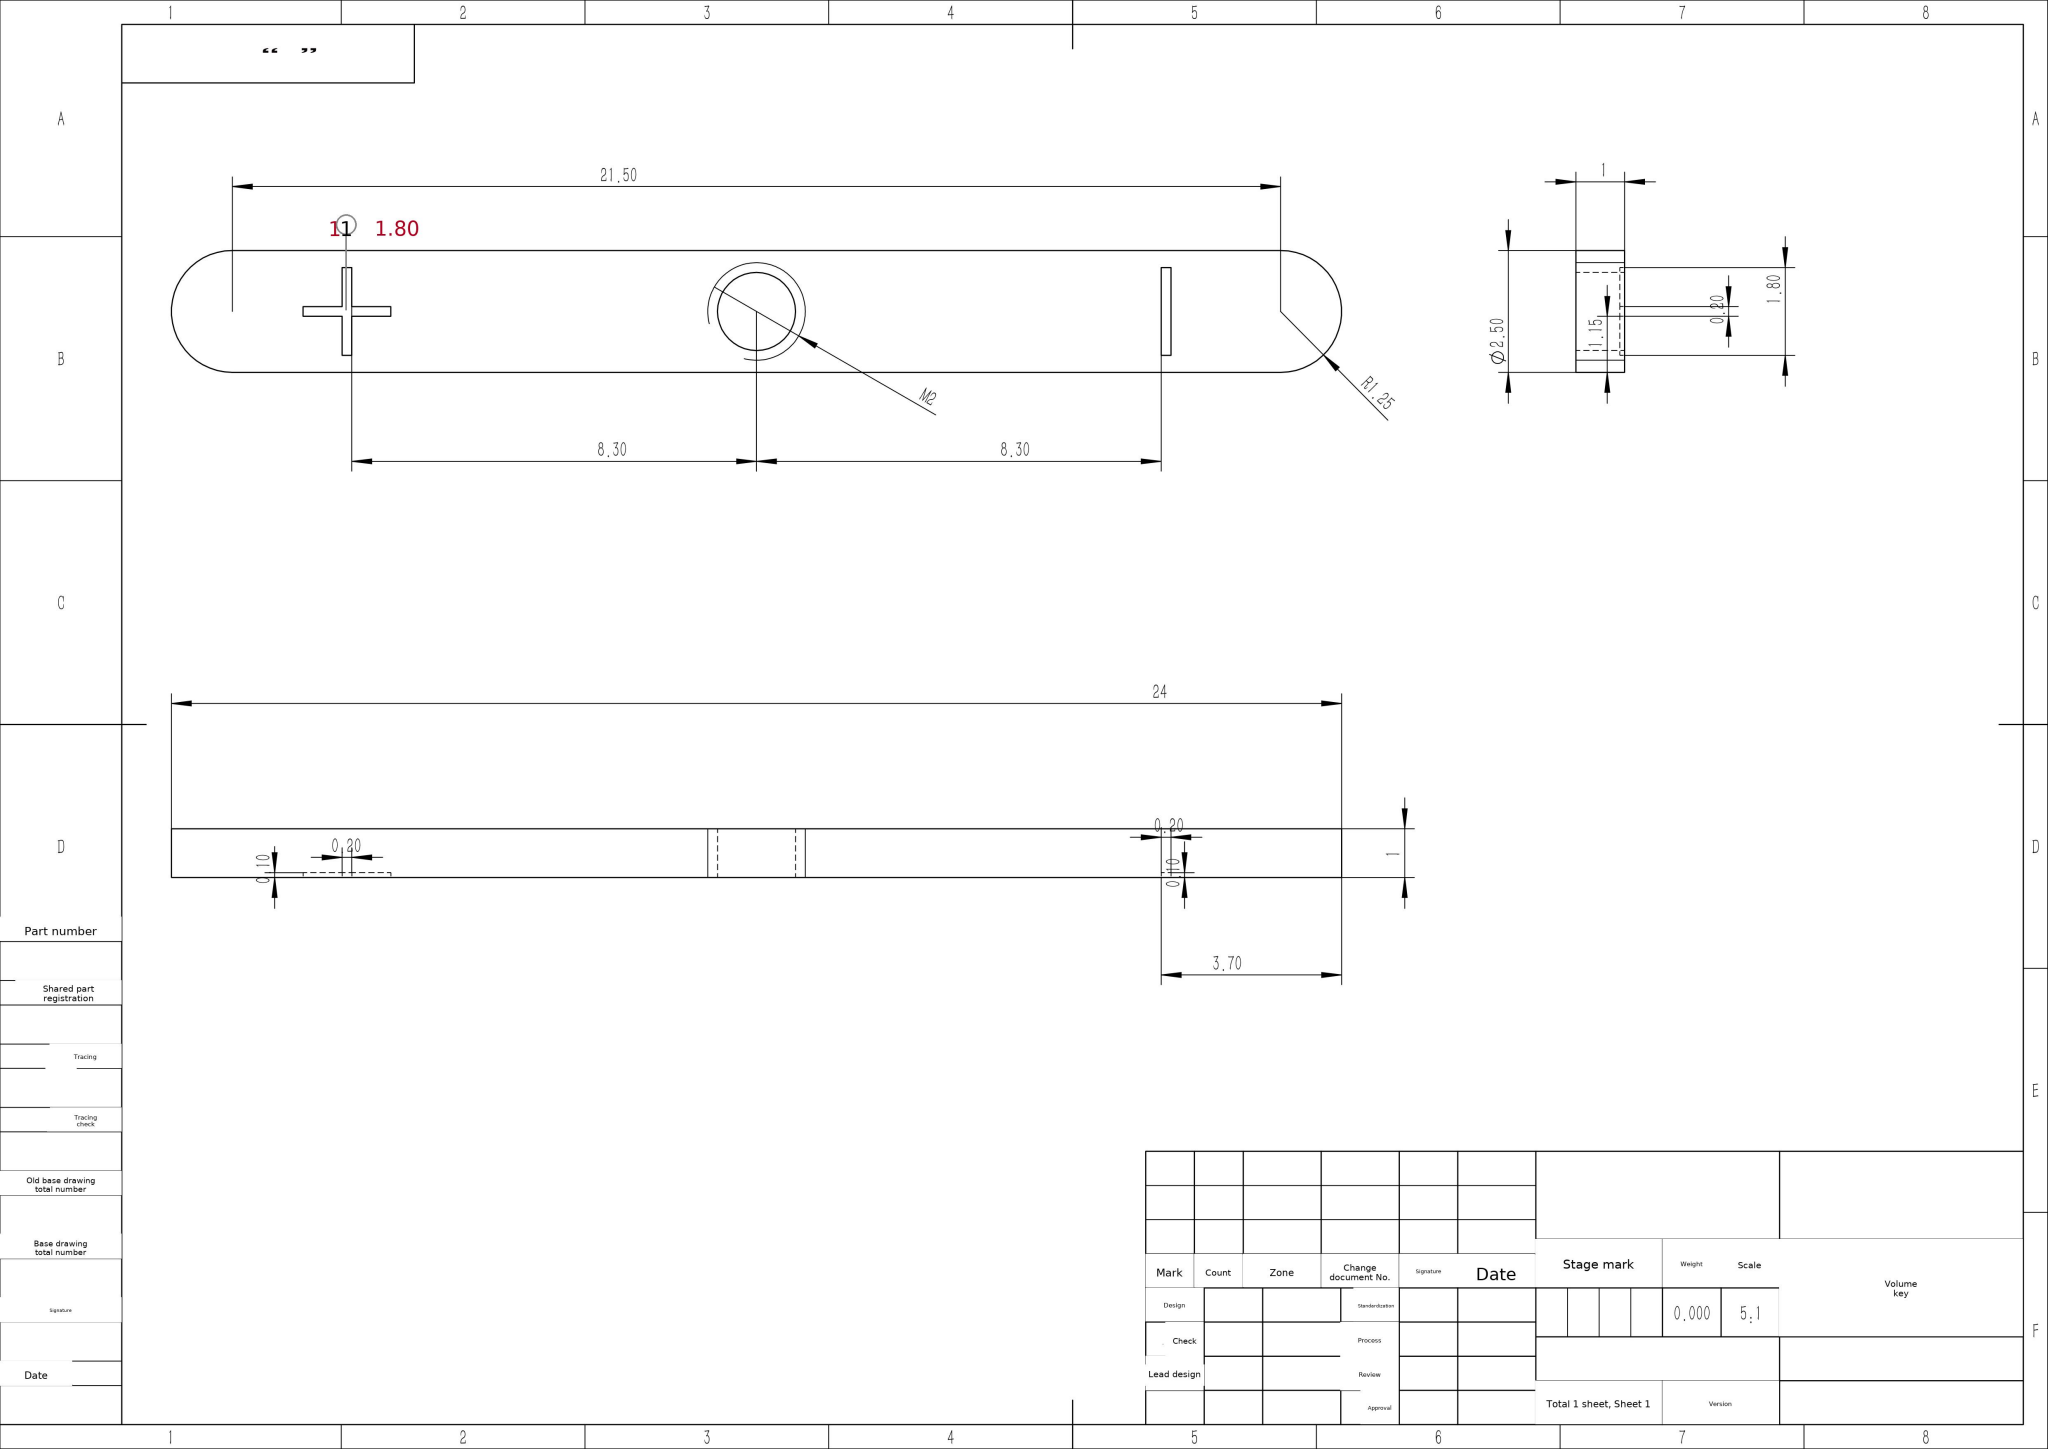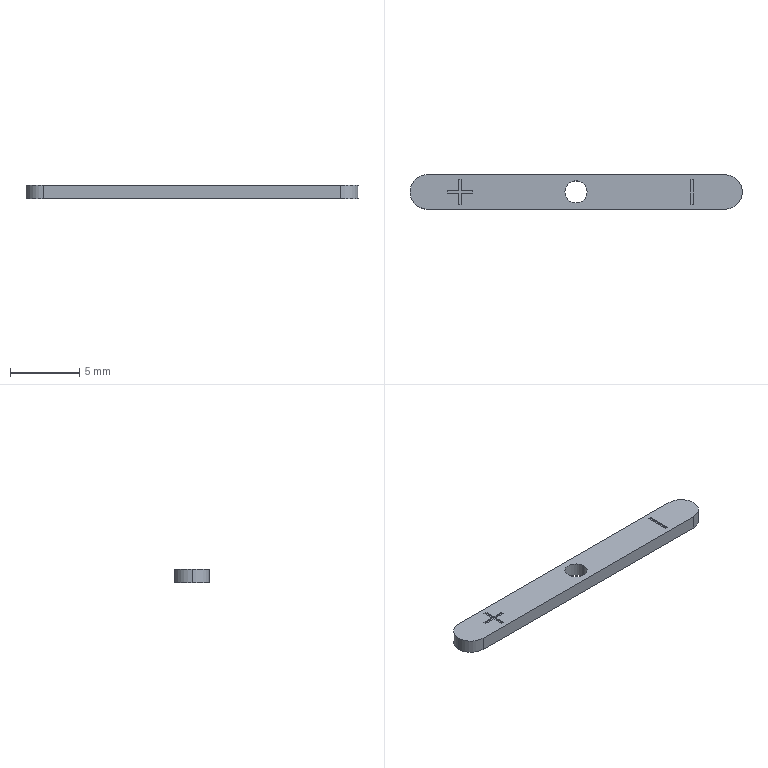Part | SolidWorks | mm | 1 solid | 27 faces | box 24 x 2.5 x 1 mm | volume 57 mm3 | plane 22 | cylinder 5 | commonest cylinder face diameters 2.5 x3 1.6 x2
build123d program:
from build123d import *

# Parameters (mm, degrees)
BOSS_EXTRUDE1_DEPTH = 1
SKETCH2_W           = 0.2
SKETCH2_H           = 1.8
SKETCH2_H_2         = 0.8
SKETCH2_W_2         = 0.8
SKETCH2_H_3         = 0.2
CUT_EXTRUDE1_DEPTH  = 0.1
M2_TAPPED_HOLE1_D   = 1.6


with BuildPart() as part:
    # Sketch1 → Boss-Extrude1 (new body)
    with BuildSketch(Plane.XY):
        with BuildLine():
            Line((-10.75, 1.25), (10.75, 1.25))
            ThreePointArc((10.75, 1.25), (12, 0), (10.75, -1.25))
            Line((10.75, -1.25), (-10.75, -1.25))
            ThreePointArc((-10.75, -1.25), (-12, 0), (-10.75, 1.25))
        make_face()
    extrude(amount=BOSS_EXTRUDE1_DEPTH)

    # Sketch2 → Cut-Extrude1 (cut)
    with BuildSketch(Plane.XY.offset(1)):
        with Locations((8.4, 0)):
            Rectangle(SKETCH2_W, SKETCH2_H)
        with Locations((-8.4, 0.5)):
            Rectangle(SKETCH2_W, SKETCH2_H_2)
        with Locations((-7.9, 0)):
            Rectangle(SKETCH2_W_2, SKETCH2_H_3)
        with Locations((-8.4, -0.5)):
            Rectangle(SKETCH2_W, SKETCH2_H_2)
        with Locations((-8.9, 0)):
            Rectangle(SKETCH2_W_2, SKETCH2_H_3)
        with Locations((-8.4, 0)):
            Rectangle(SKETCH2_W, SKETCH2_H_3)
    extrude(amount=-CUT_EXTRUDE1_DEPTH, mode=Mode.SUBTRACT)

    # M2 Tapped Hole1 (through all)
    with Locations(Plane.XY.offset(1)):
        with Locations((0, 0)):
            Hole(M2_TAPPED_HOLE1_D / 2)


solid = part.part
STEP:
#1=CARTESIAN_POINT('',(-0.8,0.,0.));
#2=VERTEX_POINT('',#1);
#3=CARTESIAN_POINT('',(0.8,0.,0.));
#4=VERTEX_POINT('',#3);
#5=CARTESIAN_POINT('',(0.,0.,0.));
#6=DIRECTION('',(0.,0.,1.));
#7=DIRECTION('',(1.,0.,0.));
#8=AXIS2_PLACEMENT_3D('',#5,#6,#7);
#9=CIRCLE('',#8,0.8);
#10=EDGE_CURVE('',#2,#4,#9,.T.);
#11=ORIENTED_EDGE('',*,*,#10,.F.);
#12=CARTESIAN_POINT('',(-0.8,0.,1.));
#13=VERTEX_POINT('',#12);
#14=CARTESIAN_POINT('',(-0.8,0.,1.));
#15=DIRECTION('',(0.,0.,1.));
#16=VECTOR('',#15,1000.);
#17=LINE('',#14,#16);
#18=EDGE_CURVE('',#2,#13,#17,.T.);
#19=ORIENTED_EDGE('',*,*,#18,.T.);
#20=CARTESIAN_POINT('',(0.8,0.,1.));
#21=VERTEX_POINT('',#20);
#22=CARTESIAN_POINT('',(0.,0.,1.));
#23=DIRECTION('',(0.,0.,1.));
#24=DIRECTION('',(1.,0.,0.));
#25=AXIS2_PLACEMENT_3D('',#22,#23,#24);
#26=CIRCLE('',#25,0.8);
#27=EDGE_CURVE('',#13,#21,#26,.T.);
#28=ORIENTED_EDGE('',*,*,#27,.T.);
#29=CARTESIAN_POINT('',(0.8,0.,1.));
#30=DIRECTION('',(0.,0.,1.));
#31=VECTOR('',#30,1000.);
#32=LINE('',#29,#31);
#33=EDGE_CURVE('',#4,#21,#32,.T.);
#34=ORIENTED_EDGE('',*,*,#33,.F.);
#35=EDGE_LOOP('',(#11,#19,#28,#34));
#36=FACE_OUTER_BOUND('',#35,.T.);
#37=CARTESIAN_POINT('',(0.,0.,1.));
#38=DIRECTION('',(0.,0.,1.));
#39=DIRECTION('',(1.,0.,0.));
#40=AXIS2_PLACEMENT_3D('',#37,#38,#39);
#41=CYLINDRICAL_SURFACE('',#40,0.8);
#42=ADVANCED_FACE('',(#36),#41,.F.);
#43=CARTESIAN_POINT('',(-12.,0.,1.));
#44=VERTEX_POINT('',#43);
#45=CARTESIAN_POINT('',(-10.75,-1.25,1.));
#46=VERTEX_POINT('',#45);
#47=CARTESIAN_POINT('',(-10.75,0.,1.));
#48=DIRECTION('',(0.,0.,1.));
#49=DIRECTION('',(1.,0.,0.));
#50=AXIS2_PLACEMENT_3D('',#47,#48,#49);
#51=CIRCLE('',#50,1.25);
#52=EDGE_CURVE('',#44,#46,#51,.T.);
#53=ORIENTED_EDGE('',*,*,#52,.F.);
#54=CARTESIAN_POINT('',(-12.,0.,0.));
#55=VERTEX_POINT('',#54);
#56=CARTESIAN_POINT('',(-12.,0.,1.));
#57=DIRECTION('',(0.,0.,-1.));
#58=VECTOR('',#57,1000.);
#59=LINE('',#56,#58);
#60=EDGE_CURVE('',#44,#55,#59,.T.);
#61=ORIENTED_EDGE('',*,*,#60,.T.);
#62=CARTESIAN_POINT('',(-10.75,-1.25,0.));
#63=VERTEX_POINT('',#62);
#64=CARTESIAN_POINT('',(-10.75,0.,0.));
#65=DIRECTION('',(0.,0.,1.));
#66=DIRECTION('',(1.,0.,0.));
#67=AXIS2_PLACEMENT_3D('',#64,#65,#66);
#68=CIRCLE('',#67,1.25);
#69=EDGE_CURVE('',#55,#63,#68,.T.);
#70=ORIENTED_EDGE('',*,*,#69,.T.);
#71=CARTESIAN_POINT('',(-10.75,-1.25,1.));
#72=DIRECTION('',(0.,0.,-1.));
#73=VECTOR('',#72,1000.);
#74=LINE('',#71,#73);
#75=EDGE_CURVE('',#46,#63,#74,.T.);
#76=ORIENTED_EDGE('',*,*,#75,.F.);
#77=EDGE_LOOP('',(#53,#61,#70,#76));
#78=FACE_OUTER_BOUND('',#77,.T.);
#79=CARTESIAN_POINT('',(-10.75,0.,1.));
#80=DIRECTION('',(0.,0.,-1.));
#81=DIRECTION('',(-1.,0.,0.));
#82=AXIS2_PLACEMENT_3D('',#79,#80,#81);
#83=CYLINDRICAL_SURFACE('',#82,1.25);
#84=ADVANCED_FACE('',(#78),#83,.T.);
#85=ORIENTED_EDGE('',*,*,#60,.F.);
#86=CARTESIAN_POINT('',(-10.75,1.25,1.));
#87=VERTEX_POINT('',#86);
#88=CARTESIAN_POINT('',(-10.75,0.,1.));
#89=DIRECTION('',(0.,0.,1.));
#90=DIRECTION('',(1.,0.,0.));
#91=AXIS2_PLACEMENT_3D('',#88,#89,#90);
#92=CIRCLE('',#91,1.25);
#93=EDGE_CURVE('',#87,#44,#92,.T.);
#94=ORIENTED_EDGE('',*,*,#93,.F.);
#95=CARTESIAN_POINT('',(-10.75,1.25,0.));
#96=VERTEX_POINT('',#95);
#97=CARTESIAN_POINT('',(-10.75,1.25,1.));
#98=DIRECTION('',(0.,0.,-1.));
#99=VECTOR('',#98,1000.);
#100=LINE('',#97,#99);
#101=EDGE_CURVE('',#87,#96,#100,.T.);
#102=ORIENTED_EDGE('',*,*,#101,.T.);
#103=CARTESIAN_POINT('',(-10.75,0.,0.));
#104=DIRECTION('',(0.,0.,1.));
#105=DIRECTION('',(1.,0.,0.));
#106=AXIS2_PLACEMENT_3D('',#103,#104,#105);
#107=CIRCLE('',#106,1.25);
#108=EDGE_CURVE('',#96,#55,#107,.T.);
#109=ORIENTED_EDGE('',*,*,#108,.T.);
#110=EDGE_LOOP('',(#85,#94,#102,#109));
#111=FACE_OUTER_BOUND('',#110,.T.);
#112=CARTESIAN_POINT('',(-10.75,0.,1.));
#113=DIRECTION('',(0.,0.,-1.));
#114=DIRECTION('',(-1.,0.,0.));
#115=AXIS2_PLACEMENT_3D('',#112,#113,#114);
#116=CYLINDRICAL_SURFACE('',#115,1.25);
#117=ADVANCED_FACE('',(#111),#116,.T.);
#118=CARTESIAN_POINT('',(10.75,-1.25,0.));
#119=VERTEX_POINT('',#118);
#120=CARTESIAN_POINT('',(-10.75,-1.25,0.));
#121=DIRECTION('',(1.,0.,0.));
#122=VECTOR('',#121,1000.);
#123=LINE('',#120,#122);
#124=EDGE_CURVE('',#63,#119,#123,.T.);
#125=ORIENTED_EDGE('',*,*,#124,.T.);
#126=CARTESIAN_POINT('',(10.75,-1.25,1.));
#127=VERTEX_POINT('',#126);
#128=CARTESIAN_POINT('',(10.75,-1.25,1.));
#129=DIRECTION('',(0.,0.,-1.));
#130=VECTOR('',#129,1000.);
#131=LINE('',#128,#130);
#132=EDGE_CURVE('',#127,#119,#131,.T.);
#133=ORIENTED_EDGE('',*,*,#132,.F.);
#134=CARTESIAN_POINT('',(-10.75,-1.25,1.));
#135=DIRECTION('',(1.,0.,0.));
#136=VECTOR('',#135,1000.);
#137=LINE('',#134,#136);
#138=EDGE_CURVE('',#46,#127,#137,.T.);
#139=ORIENTED_EDGE('',*,*,#138,.F.);
#140=ORIENTED_EDGE('',*,*,#75,.T.);
#141=EDGE_LOOP('',(#125,#133,#139,#140));
#142=FACE_OUTER_BOUND('',#141,.T.);
#143=CARTESIAN_POINT('',(-10.75,-1.25,1.));
#144=DIRECTION('',(0.,1.,0.));
#145=DIRECTION('',(0.,0.,1.));
#146=AXIS2_PLACEMENT_3D('',#143,#144,#145);
#147=PLANE('',#146);
#148=ADVANCED_FACE('',(#142),#147,.F.);
#149=CARTESIAN_POINT('',(10.75,1.25,0.));
#150=VERTEX_POINT('',#149);
#151=CARTESIAN_POINT('',(10.75,0.,0.));
#152=DIRECTION('',(0.,0.,1.));
#153=DIRECTION('',(1.,0.,0.));
#154=AXIS2_PLACEMENT_3D('',#151,#152,#153);
#155=CIRCLE('',#154,1.25);
#156=EDGE_CURVE('',#119,#150,#155,.T.);
#157=ORIENTED_EDGE('',*,*,#156,.T.);
#158=CARTESIAN_POINT('',(10.75,1.25,1.));
#159=VERTEX_POINT('',#158);
#160=CARTESIAN_POINT('',(10.75,1.25,1.));
#161=DIRECTION('',(0.,0.,-1.));
#162=VECTOR('',#161,1000.);
#163=LINE('',#160,#162);
#164=EDGE_CURVE('',#159,#150,#163,.T.);
#165=ORIENTED_EDGE('',*,*,#164,.F.);
#166=CARTESIAN_POINT('',(10.75,0.,1.));
#167=DIRECTION('',(0.,0.,1.));
#168=DIRECTION('',(1.,0.,0.));
#169=AXIS2_PLACEMENT_3D('',#166,#167,#168);
#170=CIRCLE('',#169,1.25);
#171=EDGE_CURVE('',#127,#159,#170,.T.);
#172=ORIENTED_EDGE('',*,*,#171,.F.);
#173=ORIENTED_EDGE('',*,*,#132,.T.);
#174=EDGE_LOOP('',(#157,#165,#172,#173));
#175=FACE_OUTER_BOUND('',#174,.T.);
#176=CARTESIAN_POINT('',(10.75,0.,1.));
#177=DIRECTION('',(0.,0.,-1.));
#178=DIRECTION('',(-1.,0.,0.));
#179=AXIS2_PLACEMENT_3D('',#176,#177,#178);
#180=CYLINDRICAL_SURFACE('',#179,1.25);
#181=ADVANCED_FACE('',(#175),#180,.T.);
#182=CARTESIAN_POINT('',(-10.75,1.25,0.));
#183=DIRECTION('',(-1.,0.,0.));
#184=VECTOR('',#183,1000.);
#185=LINE('',#182,#184);
#186=EDGE_CURVE('',#150,#96,#185,.T.);
#187=ORIENTED_EDGE('',*,*,#186,.T.);
#188=ORIENTED_EDGE('',*,*,#101,.F.);
#189=CARTESIAN_POINT('',(-10.75,1.25,1.));
#190=DIRECTION('',(-1.,0.,0.));
#191=VECTOR('',#190,1000.);
#192=LINE('',#189,#191);
#193=EDGE_CURVE('',#159,#87,#192,.T.);
#194=ORIENTED_EDGE('',*,*,#193,.F.);
#195=ORIENTED_EDGE('',*,*,#164,.T.);
#196=EDGE_LOOP('',(#187,#188,#194,#195));
#197=FACE_OUTER_BOUND('',#196,.T.);
#198=CARTESIAN_POINT('',(-10.75,1.25,1.));
#199=DIRECTION('',(0.,-1.,0.));
#200=DIRECTION('',(0.,0.,-1.));
#201=AXIS2_PLACEMENT_3D('',#198,#199,#200);
#202=PLANE('',#201);
#203=ADVANCED_FACE('',(#197),#202,.F.);
#204=CARTESIAN_POINT('',(0.,0.,1.));
#205=DIRECTION('',(0.,0.,1.));
#206=DIRECTION('',(1.,0.,0.));
#207=AXIS2_PLACEMENT_3D('',#204,#205,#206);
#208=CIRCLE('',#207,0.8);
#209=EDGE_CURVE('',#21,#13,#208,.T.);
#210=ORIENTED_EDGE('',*,*,#209,.F.);
#211=ORIENTED_EDGE('',*,*,#27,.F.);
#212=EDGE_LOOP('',(#210,#211));
#213=FACE_BOUND('',#212,.T.);
#214=CARTESIAN_POINT('',(8.5,0.9,1.));
#215=VERTEX_POINT('',#214);
#216=CARTESIAN_POINT('',(8.3,0.9,1.));
#217=VERTEX_POINT('',#216);
#218=CARTESIAN_POINT('',(-0.,0.9,1.));
#219=DIRECTION('',(-1.,-0.,0.));
#220=VECTOR('',#219,1000.);
#221=LINE('',#218,#220);
#222=EDGE_CURVE('',#215,#217,#221,.T.);
#223=ORIENTED_EDGE('',*,*,#222,.F.);
#224=CARTESIAN_POINT('',(8.5,-0.9,1.));
#225=VERTEX_POINT('',#224);
#226=CARTESIAN_POINT('',(8.5,-0.,1.));
#227=DIRECTION('',(-0.,-1.,0.));
#228=VECTOR('',#227,1000.);
#229=LINE('',#226,#228);
#230=EDGE_CURVE('',#215,#225,#229,.T.);
#231=ORIENTED_EDGE('',*,*,#230,.T.);
#232=CARTESIAN_POINT('',(8.3,-0.9,1.));
#233=VERTEX_POINT('',#232);
#234=CARTESIAN_POINT('',(0.,-0.9,1.));
#235=DIRECTION('',(-1.,-0.,0.));
#236=VECTOR('',#235,1000.);
#237=LINE('',#234,#236);
#238=EDGE_CURVE('',#225,#233,#237,.T.);
#239=ORIENTED_EDGE('',*,*,#238,.T.);
#240=CARTESIAN_POINT('',(8.3,0.,1.));
#241=DIRECTION('',(0.,-1.,0.));
#242=VECTOR('',#241,1000.);
#243=LINE('',#240,#242);
#244=EDGE_CURVE('',#217,#233,#243,.T.);
#245=ORIENTED_EDGE('',*,*,#244,.F.);
#246=EDGE_LOOP('',(#223,#231,#239,#245));
#247=FACE_BOUND('',#246,.T.);
#248=CARTESIAN_POINT('',(-8.5,0.9,1.));
#249=VERTEX_POINT('',#248);
#250=CARTESIAN_POINT('',(-8.5,0.1,1.));
#251=VERTEX_POINT('',#250);
#252=CARTESIAN_POINT('',(-8.5,0.,1.));
#253=DIRECTION('',(0.,-1.,0.));
#254=VECTOR('',#253,1000.);
#255=LINE('',#252,#254);
#256=EDGE_CURVE('',#249,#251,#255,.T.);
#257=ORIENTED_EDGE('',*,*,#256,.F.);
#258=CARTESIAN_POINT('',(-8.3,0.9,1.));
#259=VERTEX_POINT('',#258);
#260=CARTESIAN_POINT('',(0.,0.9,1.));
#261=DIRECTION('',(1.,0.,0.));
#262=VECTOR('',#261,1000.);
#263=LINE('',#260,#262);
#264=EDGE_CURVE('',#249,#259,#263,.T.);
#265=ORIENTED_EDGE('',*,*,#264,.T.);
#266=CARTESIAN_POINT('',(-8.3,0.1,1.));
#267=VERTEX_POINT('',#266);
#268=CARTESIAN_POINT('',(-8.3,0.,1.));
#269=DIRECTION('',(0.,-1.,0.));
#270=VECTOR('',#269,1000.);
#271=LINE('',#268,#270);
#272=EDGE_CURVE('',#259,#267,#271,.T.);
#273=ORIENTED_EDGE('',*,*,#272,.T.);
#274=CARTESIAN_POINT('',(-7.5,0.1,1.));
#275=VERTEX_POINT('',#274);
#276=CARTESIAN_POINT('',(0.,0.1,1.));
#277=DIRECTION('',(1.,0.,0.));
#278=VECTOR('',#277,1000.);
#279=LINE('',#276,#278);
#280=EDGE_CURVE('',#267,#275,#279,.T.);
#281=ORIENTED_EDGE('',*,*,#280,.T.);
#282=CARTESIAN_POINT('',(-7.5,-0.1,1.));
#283=VERTEX_POINT('',#282);
#284=CARTESIAN_POINT('',(-7.5,0.,1.));
#285=DIRECTION('',(0.,-1.,0.));
#286=VECTOR('',#285,1000.);
#287=LINE('',#284,#286);
#288=EDGE_CURVE('',#275,#283,#287,.T.);
#289=ORIENTED_EDGE('',*,*,#288,.T.);
#290=CARTESIAN_POINT('',(-8.3,-0.1,1.));
#291=VERTEX_POINT('',#290);
#292=CARTESIAN_POINT('',(0.,-0.1,1.));
#293=DIRECTION('',(1.,0.,0.));
#294=VECTOR('',#293,1000.);
#295=LINE('',#292,#294);
#296=EDGE_CURVE('',#291,#283,#295,.T.);
#297=ORIENTED_EDGE('',*,*,#296,.F.);
#298=CARTESIAN_POINT('',(-8.3,-0.9,1.));
#299=VERTEX_POINT('',#298);
#300=CARTESIAN_POINT('',(-8.3,0.,1.));
#301=DIRECTION('',(0.,-1.,0.));
#302=VECTOR('',#301,1000.);
#303=LINE('',#300,#302);
#304=EDGE_CURVE('',#291,#299,#303,.T.);
#305=ORIENTED_EDGE('',*,*,#304,.T.);
#306=CARTESIAN_POINT('',(-8.5,-0.9,1.));
#307=VERTEX_POINT('',#306);
#308=CARTESIAN_POINT('',(0.,-0.9,1.));
#309=DIRECTION('',(1.,0.,0.));
#310=VECTOR('',#309,1000.);
#311=LINE('',#308,#310);
#312=EDGE_CURVE('',#307,#299,#311,.T.);
#313=ORIENTED_EDGE('',*,*,#312,.F.);
#314=CARTESIAN_POINT('',(-8.5,-0.1,1.));
#315=VERTEX_POINT('',#314);
#316=CARTESIAN_POINT('',(-8.5,0.,1.));
#317=DIRECTION('',(0.,-1.,0.));
#318=VECTOR('',#317,1000.);
#319=LINE('',#316,#318);
#320=EDGE_CURVE('',#315,#307,#319,.T.);
#321=ORIENTED_EDGE('',*,*,#320,.F.);
#322=CARTESIAN_POINT('',(-9.3,-0.1,1.));
#323=VERTEX_POINT('',#322);
#324=CARTESIAN_POINT('',(0.,-0.1,1.));
#325=DIRECTION('',(1.,0.,0.));
#326=VECTOR('',#325,1000.);
#327=LINE('',#324,#326);
#328=EDGE_CURVE('',#323,#315,#327,.T.);
#329=ORIENTED_EDGE('',*,*,#328,.F.);
#330=CARTESIAN_POINT('',(-9.3,0.1,1.));
#331=VERTEX_POINT('',#330);
#332=CARTESIAN_POINT('',(-9.3,0.,1.));
#333=DIRECTION('',(0.,-1.,0.));
#334=VECTOR('',#333,1000.);
#335=LINE('',#332,#334);
#336=EDGE_CURVE('',#331,#323,#335,.T.);
#337=ORIENTED_EDGE('',*,*,#336,.F.);
#338=CARTESIAN_POINT('',(0.,0.1,1.));
#339=DIRECTION('',(1.,0.,0.));
#340=VECTOR('',#339,1000.);
#341=LINE('',#338,#340);
#342=EDGE_CURVE('',#331,#251,#341,.T.);
#343=ORIENTED_EDGE('',*,*,#342,.T.);
#344=EDGE_LOOP('',(#257,#265,#273,#281,#289,#297,#305,#313,#321,#329,#337,#343));
#345=FACE_BOUND('',#344,.T.);
#346=ORIENTED_EDGE('',*,*,#93,.T.);
#347=ORIENTED_EDGE('',*,*,#52,.T.);
#348=ORIENTED_EDGE('',*,*,#138,.T.);
#349=ORIENTED_EDGE('',*,*,#171,.T.);
#350=ORIENTED_EDGE('',*,*,#193,.T.);
#351=EDGE_LOOP('',(#346,#347,#348,#349,#350));
#352=FACE_OUTER_BOUND('',#351,.T.);
#353=CARTESIAN_POINT('',(-10.75,0.,1.));
#354=DIRECTION('',(0.,0.,1.));
#355=DIRECTION('',(1.,0.,0.));
#356=AXIS2_PLACEMENT_3D('',#353,#354,#355);
#357=PLANE('',#356);
#358=ADVANCED_FACE('',(#213,#247,#345,#352),#357,.T.);
#359=CARTESIAN_POINT('',(0.,0.,0.));
#360=DIRECTION('',(0.,0.,1.));
#361=DIRECTION('',(1.,0.,0.));
#362=AXIS2_PLACEMENT_3D('',#359,#360,#361);
#363=CIRCLE('',#362,0.8);
#364=EDGE_CURVE('',#4,#2,#363,.T.);
#365=ORIENTED_EDGE('',*,*,#364,.T.);
#366=ORIENTED_EDGE('',*,*,#10,.T.);
#367=EDGE_LOOP('',(#365,#366));
#368=FACE_BOUND('',#367,.T.);
#369=ORIENTED_EDGE('',*,*,#108,.F.);
#370=ORIENTED_EDGE('',*,*,#186,.F.);
#371=ORIENTED_EDGE('',*,*,#156,.F.);
#372=ORIENTED_EDGE('',*,*,#124,.F.);
#373=ORIENTED_EDGE('',*,*,#69,.F.);
#374=EDGE_LOOP('',(#369,#370,#371,#372,#373));
#375=FACE_OUTER_BOUND('',#374,.T.);
#376=CARTESIAN_POINT('',(-10.75,0.,0.));
#377=DIRECTION('',(0.,0.,1.));
#378=DIRECTION('',(1.,0.,0.));
#379=AXIS2_PLACEMENT_3D('',#376,#377,#378);
#380=PLANE('',#379);
#381=ADVANCED_FACE('',(#368,#375),#380,.F.);
#382=ORIENTED_EDGE('',*,*,#256,.T.);
#383=CARTESIAN_POINT('',(-8.5,0.1,0.9));
#384=VERTEX_POINT('',#383);
#385=CARTESIAN_POINT('',(-8.5,0.1,0.9));
#386=DIRECTION('',(0.,0.,1.));
#387=VECTOR('',#386,1000.);
#388=LINE('',#385,#387);
#389=EDGE_CURVE('',#384,#251,#388,.T.);
#390=ORIENTED_EDGE('',*,*,#389,.F.);
#391=CARTESIAN_POINT('',(-8.5,0.9,0.9));
#392=VERTEX_POINT('',#391);
#393=CARTESIAN_POINT('',(-8.5,0.,0.9));
#394=DIRECTION('',(0.,-1.,0.));
#395=VECTOR('',#394,1000.);
#396=LINE('',#393,#395);
#397=EDGE_CURVE('',#392,#384,#396,.T.);
#398=ORIENTED_EDGE('',*,*,#397,.F.);
#399=CARTESIAN_POINT('',(-8.5,0.9,0.9));
#400=DIRECTION('',(0.,0.,1.));
#401=VECTOR('',#400,1000.);
#402=LINE('',#399,#401);
#403=EDGE_CURVE('',#392,#249,#402,.T.);
#404=ORIENTED_EDGE('',*,*,#403,.T.);
#405=EDGE_LOOP('',(#382,#390,#398,#404));
#406=FACE_OUTER_BOUND('',#405,.T.);
#407=CARTESIAN_POINT('',(-8.5,0.,0.9));
#408=DIRECTION('',(-1.,0.,0.));
#409=DIRECTION('',(0.,0.,1.));
#410=AXIS2_PLACEMENT_3D('',#407,#408,#409);
#411=PLANE('',#410);
#412=ADVANCED_FACE('',(#406),#411,.F.);
#413=ORIENTED_EDGE('',*,*,#264,.F.);
#414=ORIENTED_EDGE('',*,*,#403,.F.);
#415=CARTESIAN_POINT('',(-8.3,0.9,0.9));
#416=VERTEX_POINT('',#415);
#417=CARTESIAN_POINT('',(0.,0.9,0.9));
#418=DIRECTION('',(1.,0.,0.));
#419=VECTOR('',#418,1000.);
#420=LINE('',#417,#419);
#421=EDGE_CURVE('',#392,#416,#420,.T.);
#422=ORIENTED_EDGE('',*,*,#421,.T.);
#423=CARTESIAN_POINT('',(-8.3,0.9,0.9));
#424=DIRECTION('',(0.,0.,1.));
#425=VECTOR('',#424,1000.);
#426=LINE('',#423,#425);
#427=EDGE_CURVE('',#416,#259,#426,.T.);
#428=ORIENTED_EDGE('',*,*,#427,.T.);
#429=EDGE_LOOP('',(#413,#414,#422,#428));
#430=FACE_OUTER_BOUND('',#429,.T.);
#431=CARTESIAN_POINT('',(0.,0.9,0.9));
#432=DIRECTION('',(0.,-1.,0.));
#433=DIRECTION('',(0.,0.,-1.));
#434=AXIS2_PLACEMENT_3D('',#431,#432,#433);
#435=PLANE('',#434);
#436=ADVANCED_FACE('',(#430),#435,.T.);
#437=ORIENTED_EDGE('',*,*,#272,.F.);
#438=ORIENTED_EDGE('',*,*,#427,.F.);
#439=CARTESIAN_POINT('',(-8.3,0.1,0.9));
#440=VERTEX_POINT('',#439);
#441=CARTESIAN_POINT('',(-8.3,0.,0.9));
#442=DIRECTION('',(0.,-1.,0.));
#443=VECTOR('',#442,1000.);
#444=LINE('',#441,#443);
#445=EDGE_CURVE('',#416,#440,#444,.T.);
#446=ORIENTED_EDGE('',*,*,#445,.T.);
#447=CARTESIAN_POINT('',(-8.3,0.1,0.9));
#448=DIRECTION('',(0.,0.,1.));
#449=VECTOR('',#448,1000.);
#450=LINE('',#447,#449);
#451=EDGE_CURVE('',#440,#267,#450,.T.);
#452=ORIENTED_EDGE('',*,*,#451,.T.);
#453=EDGE_LOOP('',(#437,#438,#446,#452));
#454=FACE_OUTER_BOUND('',#453,.T.);
#455=CARTESIAN_POINT('',(-8.3,0.,0.9));
#456=DIRECTION('',(-1.,0.,0.));
#457=DIRECTION('',(0.,0.,1.));
#458=AXIS2_PLACEMENT_3D('',#455,#456,#457);
#459=PLANE('',#458);
#460=ADVANCED_FACE('',(#454),#459,.T.);
#461=ORIENTED_EDGE('',*,*,#280,.F.);
#462=ORIENTED_EDGE('',*,*,#451,.F.);
#463=CARTESIAN_POINT('',(-7.5,0.1,0.9));
#464=VERTEX_POINT('',#463);
#465=CARTESIAN_POINT('',(0.,0.1,0.9));
#466=DIRECTION('',(1.,0.,0.));
#467=VECTOR('',#466,1000.);
#468=LINE('',#465,#467);
#469=EDGE_CURVE('',#440,#464,#468,.T.);
#470=ORIENTED_EDGE('',*,*,#469,.T.);
#471=CARTESIAN_POINT('',(-7.5,0.1,0.9));
#472=DIRECTION('',(0.,0.,1.));
#473=VECTOR('',#472,1000.);
#474=LINE('',#471,#473);
#475=EDGE_CURVE('',#464,#275,#474,.T.);
#476=ORIENTED_EDGE('',*,*,#475,.T.);
#477=EDGE_LOOP('',(#461,#462,#470,#476));
#478=FACE_OUTER_BOUND('',#477,.T.);
#479=CARTESIAN_POINT('',(0.,0.1,0.9));
#480=DIRECTION('',(0.,-1.,0.));
#481=DIRECTION('',(0.,0.,-1.));
#482=AXIS2_PLACEMENT_3D('',#479,#480,#481);
#483=PLANE('',#482);
#484=ADVANCED_FACE('',(#478),#483,.T.);
#485=ORIENTED_EDGE('',*,*,#288,.F.);
#486=ORIENTED_EDGE('',*,*,#475,.F.);
#487=CARTESIAN_POINT('',(-7.5,-0.1,0.9));
#488=VERTEX_POINT('',#487);
#489=CARTESIAN_POINT('',(-7.5,0.,0.9));
#490=DIRECTION('',(0.,-1.,0.));
#491=VECTOR('',#490,1000.);
#492=LINE('',#489,#491);
#493=EDGE_CURVE('',#464,#488,#492,.T.);
#494=ORIENTED_EDGE('',*,*,#493,.T.);
#495=CARTESIAN_POINT('',(-7.5,-0.1,0.9));
#496=DIRECTION('',(0.,0.,1.));
#497=VECTOR('',#496,1000.);
#498=LINE('',#495,#497);
#499=EDGE_CURVE('',#488,#283,#498,.T.);
#500=ORIENTED_EDGE('',*,*,#499,.T.);
#501=EDGE_LOOP('',(#485,#486,#494,#500));
#502=FACE_OUTER_BOUND('',#501,.T.);
#503=CARTESIAN_POINT('',(-7.5,0.,0.9));
#504=DIRECTION('',(-1.,0.,0.));
#505=DIRECTION('',(0.,0.,1.));
#506=AXIS2_PLACEMENT_3D('',#503,#504,#505);
#507=PLANE('',#506);
#508=ADVANCED_FACE('',(#502),#507,.T.);
#509=ORIENTED_EDGE('',*,*,#296,.T.);
#510=ORIENTED_EDGE('',*,*,#499,.F.);
#511=CARTESIAN_POINT('',(-8.3,-0.1,0.9));
#512=VERTEX_POINT('',#511);
#513=CARTESIAN_POINT('',(0.,-0.1,0.9));
#514=DIRECTION('',(1.,0.,0.));
#515=VECTOR('',#514,1000.);
#516=LINE('',#513,#515);
#517=EDGE_CURVE('',#512,#488,#516,.T.);
#518=ORIENTED_EDGE('',*,*,#517,.F.);
#519=CARTESIAN_POINT('',(-8.3,-0.1,0.9));
#520=DIRECTION('',(0.,0.,1.));
#521=VECTOR('',#520,1000.);
#522=LINE('',#519,#521);
#523=EDGE_CURVE('',#512,#291,#522,.T.);
#524=ORIENTED_EDGE('',*,*,#523,.T.);
#525=EDGE_LOOP('',(#509,#510,#518,#524));
#526=FACE_OUTER_BOUND('',#525,.T.);
#527=CARTESIAN_POINT('',(0.,-0.1,0.9));
#528=DIRECTION('',(0.,-1.,0.));
#529=DIRECTION('',(0.,0.,-1.));
#530=AXIS2_PLACEMENT_3D('',#527,#528,#529);
#531=PLANE('',#530);
#532=ADVANCED_FACE('',(#526),#531,.F.);
#533=ORIENTED_EDGE('',*,*,#304,.F.);
#534=ORIENTED_EDGE('',*,*,#523,.F.);
#535=CARTESIAN_POINT('',(-8.3,-0.9,0.9));
#536=VERTEX_POINT('',#535);
#537=CARTESIAN_POINT('',(-8.3,0.,0.9));
#538=DIRECTION('',(0.,-1.,0.));
#539=VECTOR('',#538,1000.);
#540=LINE('',#537,#539);
#541=EDGE_CURVE('',#512,#536,#540,.T.);
#542=ORIENTED_EDGE('',*,*,#541,.T.);
#543=CARTESIAN_POINT('',(-8.3,-0.9,0.9));
#544=DIRECTION('',(0.,0.,1.));
#545=VECTOR('',#544,1000.);
#546=LINE('',#543,#545);
#547=EDGE_CURVE('',#536,#299,#546,.T.);
#548=ORIENTED_EDGE('',*,*,#547,.T.);
#549=EDGE_LOOP('',(#533,#534,#542,#548));
#550=FACE_OUTER_BOUND('',#549,.T.);
#551=CARTESIAN_POINT('',(-8.3,0.,0.9));
#552=DIRECTION('',(-1.,0.,0.));
#553=DIRECTION('',(0.,0.,1.));
#554=AXIS2_PLACEMENT_3D('',#551,#552,#553);
#555=PLANE('',#554);
#556=ADVANCED_FACE('',(#550),#555,.T.);
#557=ORIENTED_EDGE('',*,*,#312,.T.);
#558=ORIENTED_EDGE('',*,*,#547,.F.);
#559=CARTESIAN_POINT('',(-8.5,-0.9,0.9));
#560=VERTEX_POINT('',#559);
#561=CARTESIAN_POINT('',(0.,-0.9,0.9));
#562=DIRECTION('',(1.,0.,0.));
#563=VECTOR('',#562,1000.);
#564=LINE('',#561,#563);
#565=EDGE_CURVE('',#560,#536,#564,.T.);
#566=ORIENTED_EDGE('',*,*,#565,.F.);
#567=CARTESIAN_POINT('',(-8.5,-0.9,0.9));
#568=DIRECTION('',(0.,0.,1.));
#569=VECTOR('',#568,1000.);
#570=LINE('',#567,#569);
#571=EDGE_CURVE('',#560,#307,#570,.T.);
#572=ORIENTED_EDGE('',*,*,#571,.T.);
#573=EDGE_LOOP('',(#557,#558,#566,#572));
#574=FACE_OUTER_BOUND('',#573,.T.);
#575=CARTESIAN_POINT('',(0.,-0.9,0.9));
#576=DIRECTION('',(0.,-1.,0.));
#577=DIRECTION('',(0.,0.,-1.));
#578=AXIS2_PLACEMENT_3D('',#575,#576,#577);
#579=PLANE('',#578);
#580=ADVANCED_FACE('',(#574),#579,.F.);
#581=ORIENTED_EDGE('',*,*,#320,.T.);
#582=ORIENTED_EDGE('',*,*,#571,.F.);
#583=CARTESIAN_POINT('',(-8.5,-0.1,0.9));
#584=VERTEX_POINT('',#583);
#585=CARTESIAN_POINT('',(-8.5,0.,0.9));
#586=DIRECTION('',(0.,-1.,0.));
#587=VECTOR('',#586,1000.);
#588=LINE('',#585,#587);
#589=EDGE_CURVE('',#584,#560,#588,.T.);
#590=ORIENTED_EDGE('',*,*,#589,.F.);
#591=CARTESIAN_POINT('',(-8.5,-0.1,0.9));
#592=DIRECTION('',(0.,0.,1.));
#593=VECTOR('',#592,1000.);
#594=LINE('',#591,#593);
#595=EDGE_CURVE('',#584,#315,#594,.T.);
#596=ORIENTED_EDGE('',*,*,#595,.T.);
#597=EDGE_LOOP('',(#581,#582,#590,#596));
#598=FACE_OUTER_BOUND('',#597,.T.);
#599=CARTESIAN_POINT('',(-8.5,0.,0.9));
#600=DIRECTION('',(-1.,0.,0.));
#601=DIRECTION('',(0.,0.,1.));
#602=AXIS2_PLACEMENT_3D('',#599,#600,#601);
#603=PLANE('',#602);
#604=ADVANCED_FACE('',(#598),#603,.F.);
#605=ORIENTED_EDGE('',*,*,#328,.T.);
#606=ORIENTED_EDGE('',*,*,#595,.F.);
#607=CARTESIAN_POINT('',(-9.3,-0.1,0.9));
#608=VERTEX_POINT('',#607);
#609=CARTESIAN_POINT('',(0.,-0.1,0.9));
#610=DIRECTION('',(1.,0.,0.));
#611=VECTOR('',#610,1000.);
#612=LINE('',#609,#611);
#613=EDGE_CURVE('',#608,#584,#612,.T.);
#614=ORIENTED_EDGE('',*,*,#613,.F.);
#615=CARTESIAN_POINT('',(-9.3,-0.1,0.9));
#616=DIRECTION('',(0.,0.,1.));
#617=VECTOR('',#616,1000.);
#618=LINE('',#615,#617);
#619=EDGE_CURVE('',#608,#323,#618,.T.);
#620=ORIENTED_EDGE('',*,*,#619,.T.);
#621=EDGE_LOOP('',(#605,#606,#614,#620));
#622=FACE_OUTER_BOUND('',#621,.T.);
#623=CARTESIAN_POINT('',(0.,-0.1,0.9));
#624=DIRECTION('',(0.,-1.,0.));
#625=DIRECTION('',(0.,0.,-1.));
#626=AXIS2_PLACEMENT_3D('',#623,#624,#625);
#627=PLANE('',#626);
#628=ADVANCED_FACE('',(#622),#627,.F.);
#629=ORIENTED_EDGE('',*,*,#336,.T.);
#630=ORIENTED_EDGE('',*,*,#619,.F.);
#631=CARTESIAN_POINT('',(-9.3,0.1,0.9));
#632=VERTEX_POINT('',#631);
#633=CARTESIAN_POINT('',(-9.3,0.,0.9));
#634=DIRECTION('',(0.,-1.,0.));
#635=VECTOR('',#634,1000.);
#636=LINE('',#633,#635);
#637=EDGE_CURVE('',#632,#608,#636,.T.);
#638=ORIENTED_EDGE('',*,*,#637,.F.);
#639=CARTESIAN_POINT('',(-9.3,0.1,0.9));
#640=DIRECTION('',(0.,0.,1.));
#641=VECTOR('',#640,1000.);
#642=LINE('',#639,#641);
#643=EDGE_CURVE('',#632,#331,#642,.T.);
#644=ORIENTED_EDGE('',*,*,#643,.T.);
#645=EDGE_LOOP('',(#629,#630,#638,#644));
#646=FACE_OUTER_BOUND('',#645,.T.);
#647=CARTESIAN_POINT('',(-9.3,0.,0.9));
#648=DIRECTION('',(-1.,0.,0.));
#649=DIRECTION('',(0.,0.,1.));
#650=AXIS2_PLACEMENT_3D('',#647,#648,#649);
#651=PLANE('',#650);
#652=ADVANCED_FACE('',(#646),#651,.F.);
#653=ORIENTED_EDGE('',*,*,#342,.F.);
#654=ORIENTED_EDGE('',*,*,#643,.F.);
#655=CARTESIAN_POINT('',(0.,0.1,0.9));
#656=DIRECTION('',(1.,0.,0.));
#657=VECTOR('',#656,1000.);
#658=LINE('',#655,#657);
#659=EDGE_CURVE('',#632,#384,#658,.T.);
#660=ORIENTED_EDGE('',*,*,#659,.T.);
#661=ORIENTED_EDGE('',*,*,#389,.T.);
#662=EDGE_LOOP('',(#653,#654,#660,#661));
#663=FACE_OUTER_BOUND('',#662,.T.);
#664=CARTESIAN_POINT('',(0.,0.1,0.9));
#665=DIRECTION('',(0.,-1.,0.));
#666=DIRECTION('',(0.,0.,-1.));
#667=AXIS2_PLACEMENT_3D('',#664,#665,#666);
#668=PLANE('',#667);
#669=ADVANCED_FACE('',(#663),#668,.T.);
#670=ORIENTED_EDGE('',*,*,#397,.T.);
#671=ORIENTED_EDGE('',*,*,#659,.F.);
#672=ORIENTED_EDGE('',*,*,#637,.T.);
#673=ORIENTED_EDGE('',*,*,#613,.T.);
#674=ORIENTED_EDGE('',*,*,#589,.T.);
#675=ORIENTED_EDGE('',*,*,#565,.T.);
#676=ORIENTED_EDGE('',*,*,#541,.F.);
#677=ORIENTED_EDGE('',*,*,#517,.T.);
#678=ORIENTED_EDGE('',*,*,#493,.F.);
#679=ORIENTED_EDGE('',*,*,#469,.F.);
#680=ORIENTED_EDGE('',*,*,#445,.F.);
#681=ORIENTED_EDGE('',*,*,#421,.F.);
#682=EDGE_LOOP('',(#670,#671,#672,#673,#674,#675,#676,#677,#678,#679,#680,#681));
#683=FACE_OUTER_BOUND('',#682,.T.);
#684=CARTESIAN_POINT('',(0.,0.,0.9));
#685=DIRECTION('',(0.,0.,1.));
#686=DIRECTION('',(1.,0.,0.));
#687=AXIS2_PLACEMENT_3D('',#684,#685,#686);
#688=PLANE('',#687);
#689=ADVANCED_FACE('',(#683),#688,.T.);
#690=ORIENTED_EDGE('',*,*,#222,.T.);
#691=CARTESIAN_POINT('',(8.3,0.9,0.9));
#692=VERTEX_POINT('',#691);
#693=CARTESIAN_POINT('',(8.3,0.9,0.9));
#694=DIRECTION('',(0.,0.,1.));
#695=VECTOR('',#694,1000.);
#696=LINE('',#693,#695);
#697=EDGE_CURVE('',#692,#217,#696,.T.);
#698=ORIENTED_EDGE('',*,*,#697,.F.);
#699=CARTESIAN_POINT('',(8.5,0.9,0.9));
#700=VERTEX_POINT('',#699);
#701=CARTESIAN_POINT('',(-0.,0.9,0.9));
#702=DIRECTION('',(-1.,-0.,0.));
#703=VECTOR('',#702,1000.);
#704=LINE('',#701,#703);
#705=EDGE_CURVE('',#700,#692,#704,.T.);
#706=ORIENTED_EDGE('',*,*,#705,.F.);
#707=CARTESIAN_POINT('',(8.5,0.9,0.9));
#708=DIRECTION('',(0.,0.,1.));
#709=VECTOR('',#708,1000.);
#710=LINE('',#707,#709);
#711=EDGE_CURVE('',#700,#215,#710,.T.);
#712=ORIENTED_EDGE('',*,*,#711,.T.);
#713=EDGE_LOOP('',(#690,#698,#706,#712));
#714=FACE_OUTER_BOUND('',#713,.T.);
#715=CARTESIAN_POINT('',(-0.,0.9,0.9));
#716=DIRECTION('',(-0.,1.,0.));
#717=DIRECTION('',(-1.,-0.,0.));
#718=AXIS2_PLACEMENT_3D('',#715,#716,#717);
#719=PLANE('',#718);
#720=ADVANCED_FACE('',(#714),#719,.F.);
#721=ORIENTED_EDGE('',*,*,#230,.F.);
#722=ORIENTED_EDGE('',*,*,#711,.F.);
#723=CARTESIAN_POINT('',(8.5,-0.9,0.9));
#724=VERTEX_POINT('',#723);
#725=CARTESIAN_POINT('',(8.5,-0.,0.9));
#726=DIRECTION('',(-0.,-1.,0.));
#727=VECTOR('',#726,1000.);
#728=LINE('',#725,#727);
#729=EDGE_CURVE('',#700,#724,#728,.T.);
#730=ORIENTED_EDGE('',*,*,#729,.T.);
#731=CARTESIAN_POINT('',(8.5,-0.9,0.9));
#732=DIRECTION('',(0.,0.,1.));
#733=VECTOR('',#732,1000.);
#734=LINE('',#731,#733);
#735=EDGE_CURVE('',#724,#225,#734,.T.);
#736=ORIENTED_EDGE('',*,*,#735,.T.);
#737=EDGE_LOOP('',(#721,#722,#730,#736));
#738=FACE_OUTER_BOUND('',#737,.T.);
#739=CARTESIAN_POINT('',(8.5,-0.,0.9));
#740=DIRECTION('',(-1.,0.,0.));
#741=DIRECTION('',(-0.,-1.,0.));
#742=AXIS2_PLACEMENT_3D('',#739,#740,#741);
#743=PLANE('',#742);
#744=ADVANCED_FACE('',(#738),#743,.T.);
#745=ORIENTED_EDGE('',*,*,#238,.F.);
#746=ORIENTED_EDGE('',*,*,#735,.F.);
#747=CARTESIAN_POINT('',(8.3,-0.9,0.9));
#748=VERTEX_POINT('',#747);
#749=CARTESIAN_POINT('',(0.,-0.9,0.9));
#750=DIRECTION('',(-1.,-0.,0.));
#751=VECTOR('',#750,1000.);
#752=LINE('',#749,#751);
#753=EDGE_CURVE('',#724,#748,#752,.T.);
#754=ORIENTED_EDGE('',*,*,#753,.T.);
#755=CARTESIAN_POINT('',(8.3,-0.9,0.9));
#756=DIRECTION('',(0.,0.,1.));
#757=VECTOR('',#756,1000.);
#758=LINE('',#755,#757);
#759=EDGE_CURVE('',#748,#233,#758,.T.);
#760=ORIENTED_EDGE('',*,*,#759,.T.);
#761=EDGE_LOOP('',(#745,#746,#754,#760));
#762=FACE_OUTER_BOUND('',#761,.T.);
#763=CARTESIAN_POINT('',(0.,-0.9,0.9));
#764=DIRECTION('',(-0.,1.,0.));
#765=DIRECTION('',(-1.,-0.,0.));
#766=AXIS2_PLACEMENT_3D('',#763,#764,#765);
#767=PLANE('',#766);
#768=ADVANCED_FACE('',(#762),#767,.T.);
#769=ORIENTED_EDGE('',*,*,#244,.T.);
#770=ORIENTED_EDGE('',*,*,#759,.F.);
#771=CARTESIAN_POINT('',(8.3,0.,0.9));
#772=DIRECTION('',(0.,-1.,0.));
#773=VECTOR('',#772,1000.);
#774=LINE('',#771,#773);
#775=EDGE_CURVE('',#692,#748,#774,.T.);
#776=ORIENTED_EDGE('',*,*,#775,.F.);
#777=ORIENTED_EDGE('',*,*,#697,.T.);
#778=EDGE_LOOP('',(#769,#770,#776,#777));
#779=FACE_OUTER_BOUND('',#778,.T.);
#780=CARTESIAN_POINT('',(8.3,0.,0.9));
#781=DIRECTION('',(-1.,0.,0.));
#782=DIRECTION('',(0.,0.,1.));
#783=AXIS2_PLACEMENT_3D('',#780,#781,#782);
#784=PLANE('',#783);
#785=ADVANCED_FACE('',(#779),#784,.F.);
#786=ORIENTED_EDGE('',*,*,#705,.T.);
#787=ORIENTED_EDGE('',*,*,#775,.T.);
#788=ORIENTED_EDGE('',*,*,#753,.F.);
#789=ORIENTED_EDGE('',*,*,#729,.F.);
#790=EDGE_LOOP('',(#786,#787,#788,#789));
#791=FACE_OUTER_BOUND('',#790,.T.);
#792=CARTESIAN_POINT('',(0.,0.,0.9));
#793=DIRECTION('',(0.,0.,1.));
#794=DIRECTION('',(1.,0.,0.));
#795=AXIS2_PLACEMENT_3D('',#792,#793,#794);
#796=PLANE('',#795);
#797=ADVANCED_FACE('',(#791),#796,.T.);
#798=ORIENTED_EDGE('',*,*,#18,.F.);
#799=ORIENTED_EDGE('',*,*,#364,.F.);
#800=ORIENTED_EDGE('',*,*,#33,.T.);
#801=ORIENTED_EDGE('',*,*,#209,.T.);
#802=EDGE_LOOP('',(#798,#799,#800,#801));
#803=FACE_OUTER_BOUND('',#802,.T.);
#804=CARTESIAN_POINT('',(0.,0.,1.));
#805=DIRECTION('',(0.,0.,1.));
#806=DIRECTION('',(1.,0.,0.));
#807=AXIS2_PLACEMENT_3D('',#804,#805,#806);
#808=CYLINDRICAL_SURFACE('',#807,0.8);
#809=ADVANCED_FACE('',(#803),#808,.F.);
#810=CLOSED_SHELL('',(#42,#84,#117,#148,#181,#203,#358,#381,#412,#436,#460,#484,#508,#532,#556,#580,#604,#628,#652,#669,#689,#720,#744,#768,#785,#797,#809));
#811=MANIFOLD_SOLID_BREP('',#810);
#812=CARTESIAN_POINT('',(0.,0.,0.));
#813=DIRECTION('',(0.,0.,1.));
#814=DIRECTION('',(1.,0.,0.));
#815=AXIS2_PLACEMENT_3D('',#812,#813,#814);
#816=(LENGTH_UNIT()NAMED_UNIT(*)SI_UNIT(.MILLI.,.METRE.));
#817=UNCERTAINTY_MEASURE_WITH_UNIT(LENGTH_MEASURE(0.00001),#816,'','');
#818=(NAMED_UNIT(*)PLANE_ANGLE_UNIT()SI_UNIT($,.RADIAN.));
#819=(NAMED_UNIT(*)SI_UNIT($,.STERADIAN.)SOLID_ANGLE_UNIT());
#820=(GEOMETRIC_REPRESENTATION_CONTEXT(3)GLOBAL_UNCERTAINTY_ASSIGNED_CONTEXT((#817))GLOBAL_UNIT_ASSIGNED_CONTEXT((#816,#818,#819))REPRESENTATION_CONTEXT('',''));
#821=ADVANCED_BREP_SHAPE_REPRESENTATION('',(#811,#815),#820);